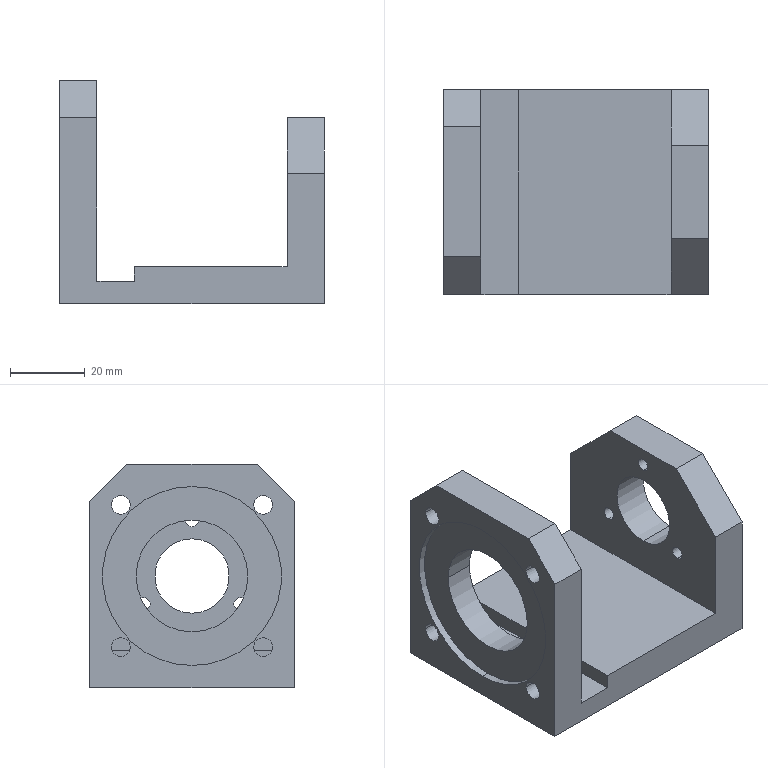Component | SolidWorks | LowerSideBeltXG-XG1-1_EncoderMount-1 | 1 solid | 37 faces | box 71 x 55 x 60 mm | volume 69610 mm3 | cylinder 20 | plane 17 | commonest cylinder face diameters 5 x8 3.5 x6 20 x2 48 x2 30 x2
build123d program:
from build123d import *

# Parameters (mm, degrees)
BOSS_EXTRUDE1_DEPTH = 27.5
SKETCH2_R           = 15
CUT_EXTRUDE1_DEPTH  = 84.53
SKETCH3_R           = 24
CUT_EXTRUDE2_DEPTH  = 2
CHAMFER1_SIZE       = 15
CHAMFER2_SIZE       = 10
SKETCH4_R           = 2.5
CUT_EXTRUDE3_DEPTH  = 84.53
SKETCH5_W           = 10
SKETCH5_H           = 55
CUT_EXTRUDE4_DEPTH  = 4
SKETCH7_R           = 10
CUT_EXTRUDE6_DEPTH  = 84.53
SKETCH8_R           = 1.75
CUT_EXTRUDE7_DEPTH  = 10


with BuildPart() as part:
    # Sketch1 → Boss-Extrude1 (new, symmetric)
    with BuildSketch(Plane.XY):
        Polygon((0, 0), (51, 0), (51, 50), (61, 50), (61, -10), (-10, -10), (-10, 40), (0, 40), align=None)
    extrude(amount=BOSS_EXTRUDE1_DEPTH, both=True)

    # Sketch2 → Cut-Extrude1 (cut, through all)
    with BuildSketch(Plane.ZY.offset(-51)):
        with Locations((0, 20)):
            Circle(SKETCH2_R)
    extrude(amount=-CUT_EXTRUDE1_DEPTH, mode=Mode.SUBTRACT)

    # Sketch3 → Cut-Extrude2 (cut)
    with BuildSketch(Plane(origin=(61, 0, 0), x_dir=(0, 0, -1), z_dir=(1, 0, 0))):
        with Locations(Location((0, 20, 0), (0, 0, 90))):
            Circle(SKETCH3_R)
    extrude(amount=-CUT_EXTRUDE2_DEPTH, mode=Mode.SUBTRACT)

    # Chamfer1
    chamfer1_edges = [part.edges().sort_by_distance(p)[0] for p in [
        (-5, 40, -27.5),
        (-5, 40, 27.5),
    ]]
    chamfer(chamfer1_edges, length=CHAMFER1_SIZE)

    # Chamfer2
    chamfer2_edges = [part.edges().sort_by_distance(p)[0] for p in [
        (56, 50, 27.5),
        (56, 50, -27.5),
    ]]
    chamfer(chamfer2_edges, length=CHAMFER2_SIZE)

    # Sketch4 → Cut-Extrude3 (cut, through all)
    with BuildSketch(Plane.ZY.offset(-51)):
        with Locations((-19.092, 39.092)):
            Circle(SKETCH4_R)
        with Locations(Location((19.092, 39.092, 0), (0, 0, 180))):
            Circle(SKETCH4_R)
        with Locations((-19.092, 0.9081)):
            Circle(SKETCH4_R)
        with Locations((19.092, 0.9081)):
            Circle(SKETCH4_R)
    extrude(amount=-CUT_EXTRUDE3_DEPTH, mode=Mode.SUBTRACT)

    # Sketch5 → Cut-Extrude4 (cut)
    with BuildSketch(Plane(origin=(0, 0, 0), x_dir=(1, 0, 0), z_dir=(0, 1, 0))):
        with Locations((46, 0)):
            Rectangle(SKETCH5_W, SKETCH5_H)
    extrude(amount=-CUT_EXTRUDE4_DEPTH, mode=Mode.SUBTRACT)

    # Sketch7 → Cut-Extrude6 (cut, through all)
    with BuildSketch(Plane(origin=(0, 0, 0), x_dir=(0, 0, -1), z_dir=(1, 0, 0))):
        with Locations(Location((0, 20, 0), (0, 0, 90))):
            Circle(SKETCH7_R)
    extrude(amount=-CUT_EXTRUDE6_DEPTH, mode=Mode.SUBTRACT)

    # Sketch8 → Cut-Extrude7 (cut)
    with BuildSketch(Plane.ZY.offset(10)):
        with Locations(Location((0, 35, 0), (0, 0, 270))):
            Circle(SKETCH8_R)
        with Locations(Location((-12.99, 12.5, 0), (0, 0, 270))):
            Circle(SKETCH8_R)
        with Locations(Location((12.99, 12.5, 0), (0, 0, 270))):
            Circle(SKETCH8_R)
    extrude(amount=-CUT_EXTRUDE7_DEPTH, mode=Mode.SUBTRACT)


solid = part.part

# Placed as in the assembly
solid = solid.moved(Location((-123.22, 625, 94), (-90, 0, 180)))